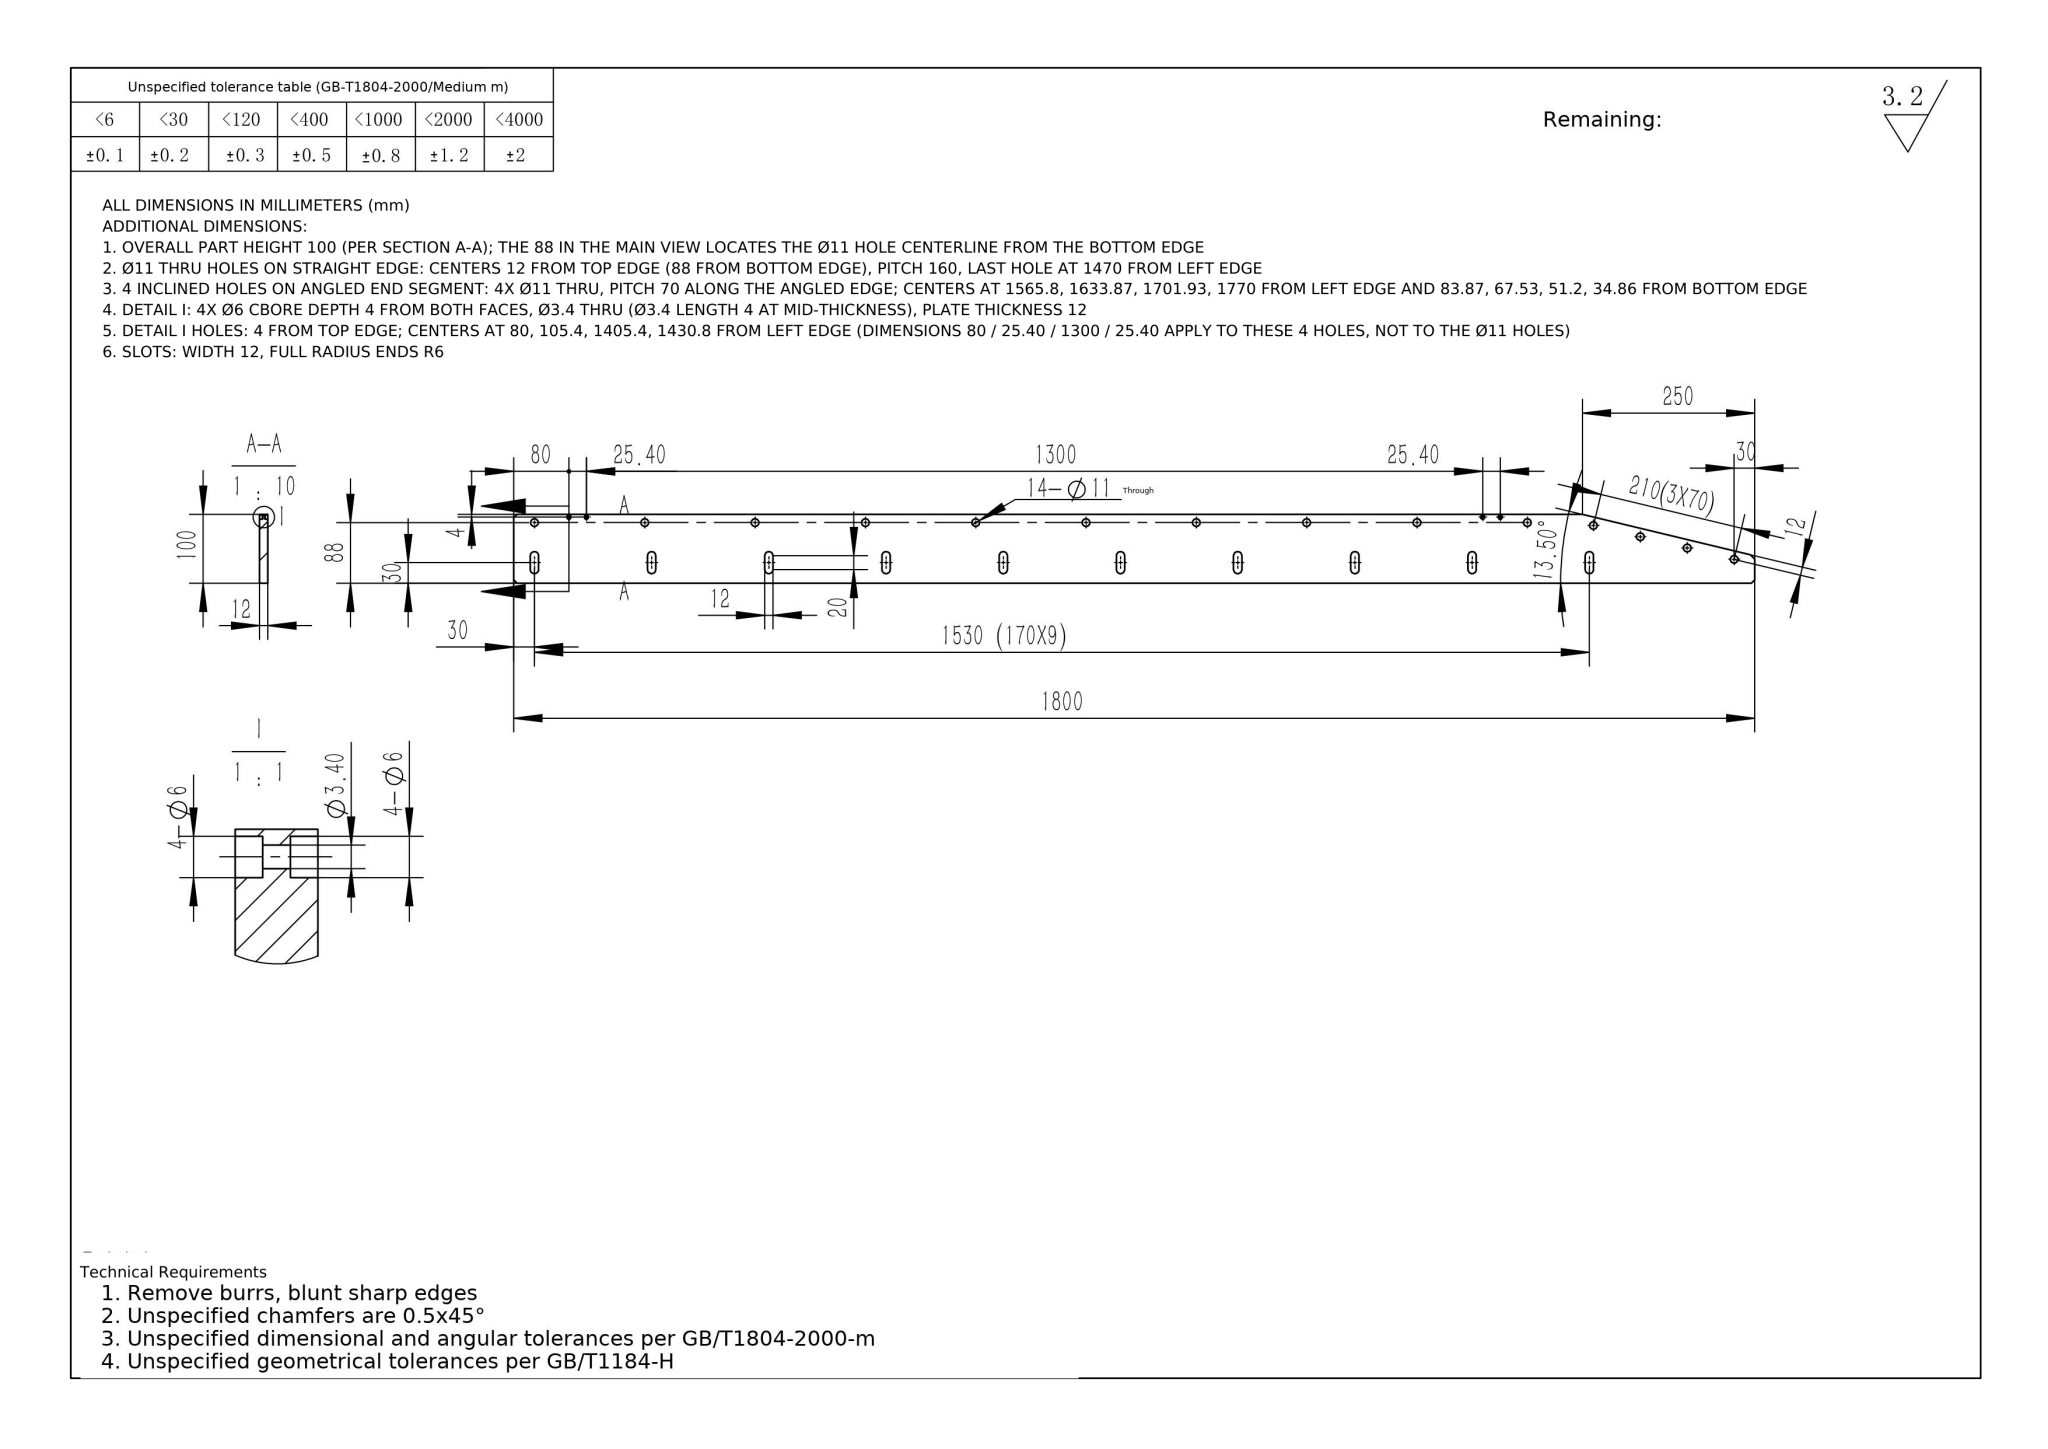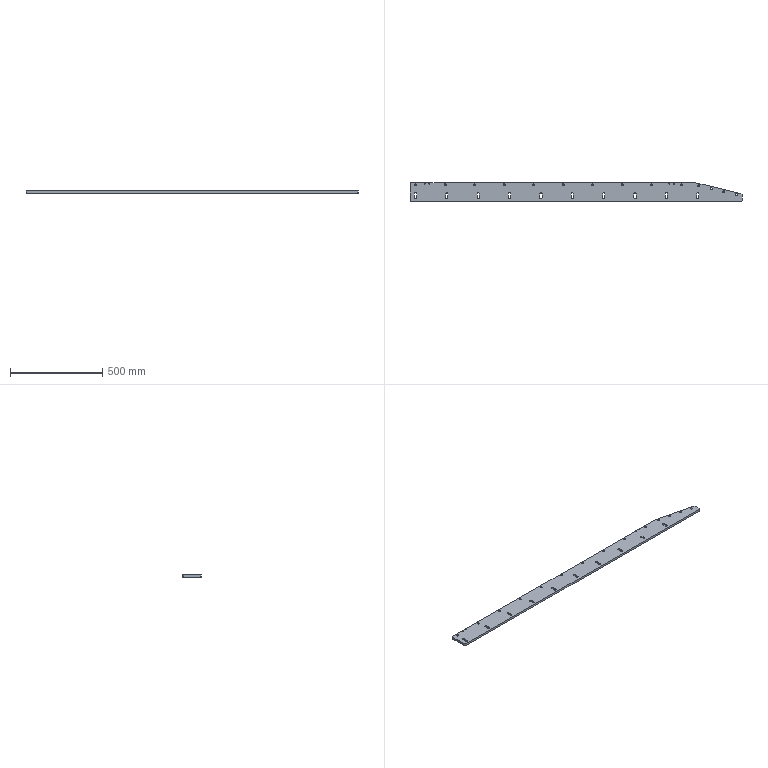Part | NX | mm | 1 solid | 111 faces | box 1800 x 100 x 12 mm | volume 2009965 mm3 | cylinder 72 | plane 39 | commonest cylinder face diameters 11 x28 12 x20 6 x16 3.4 x8